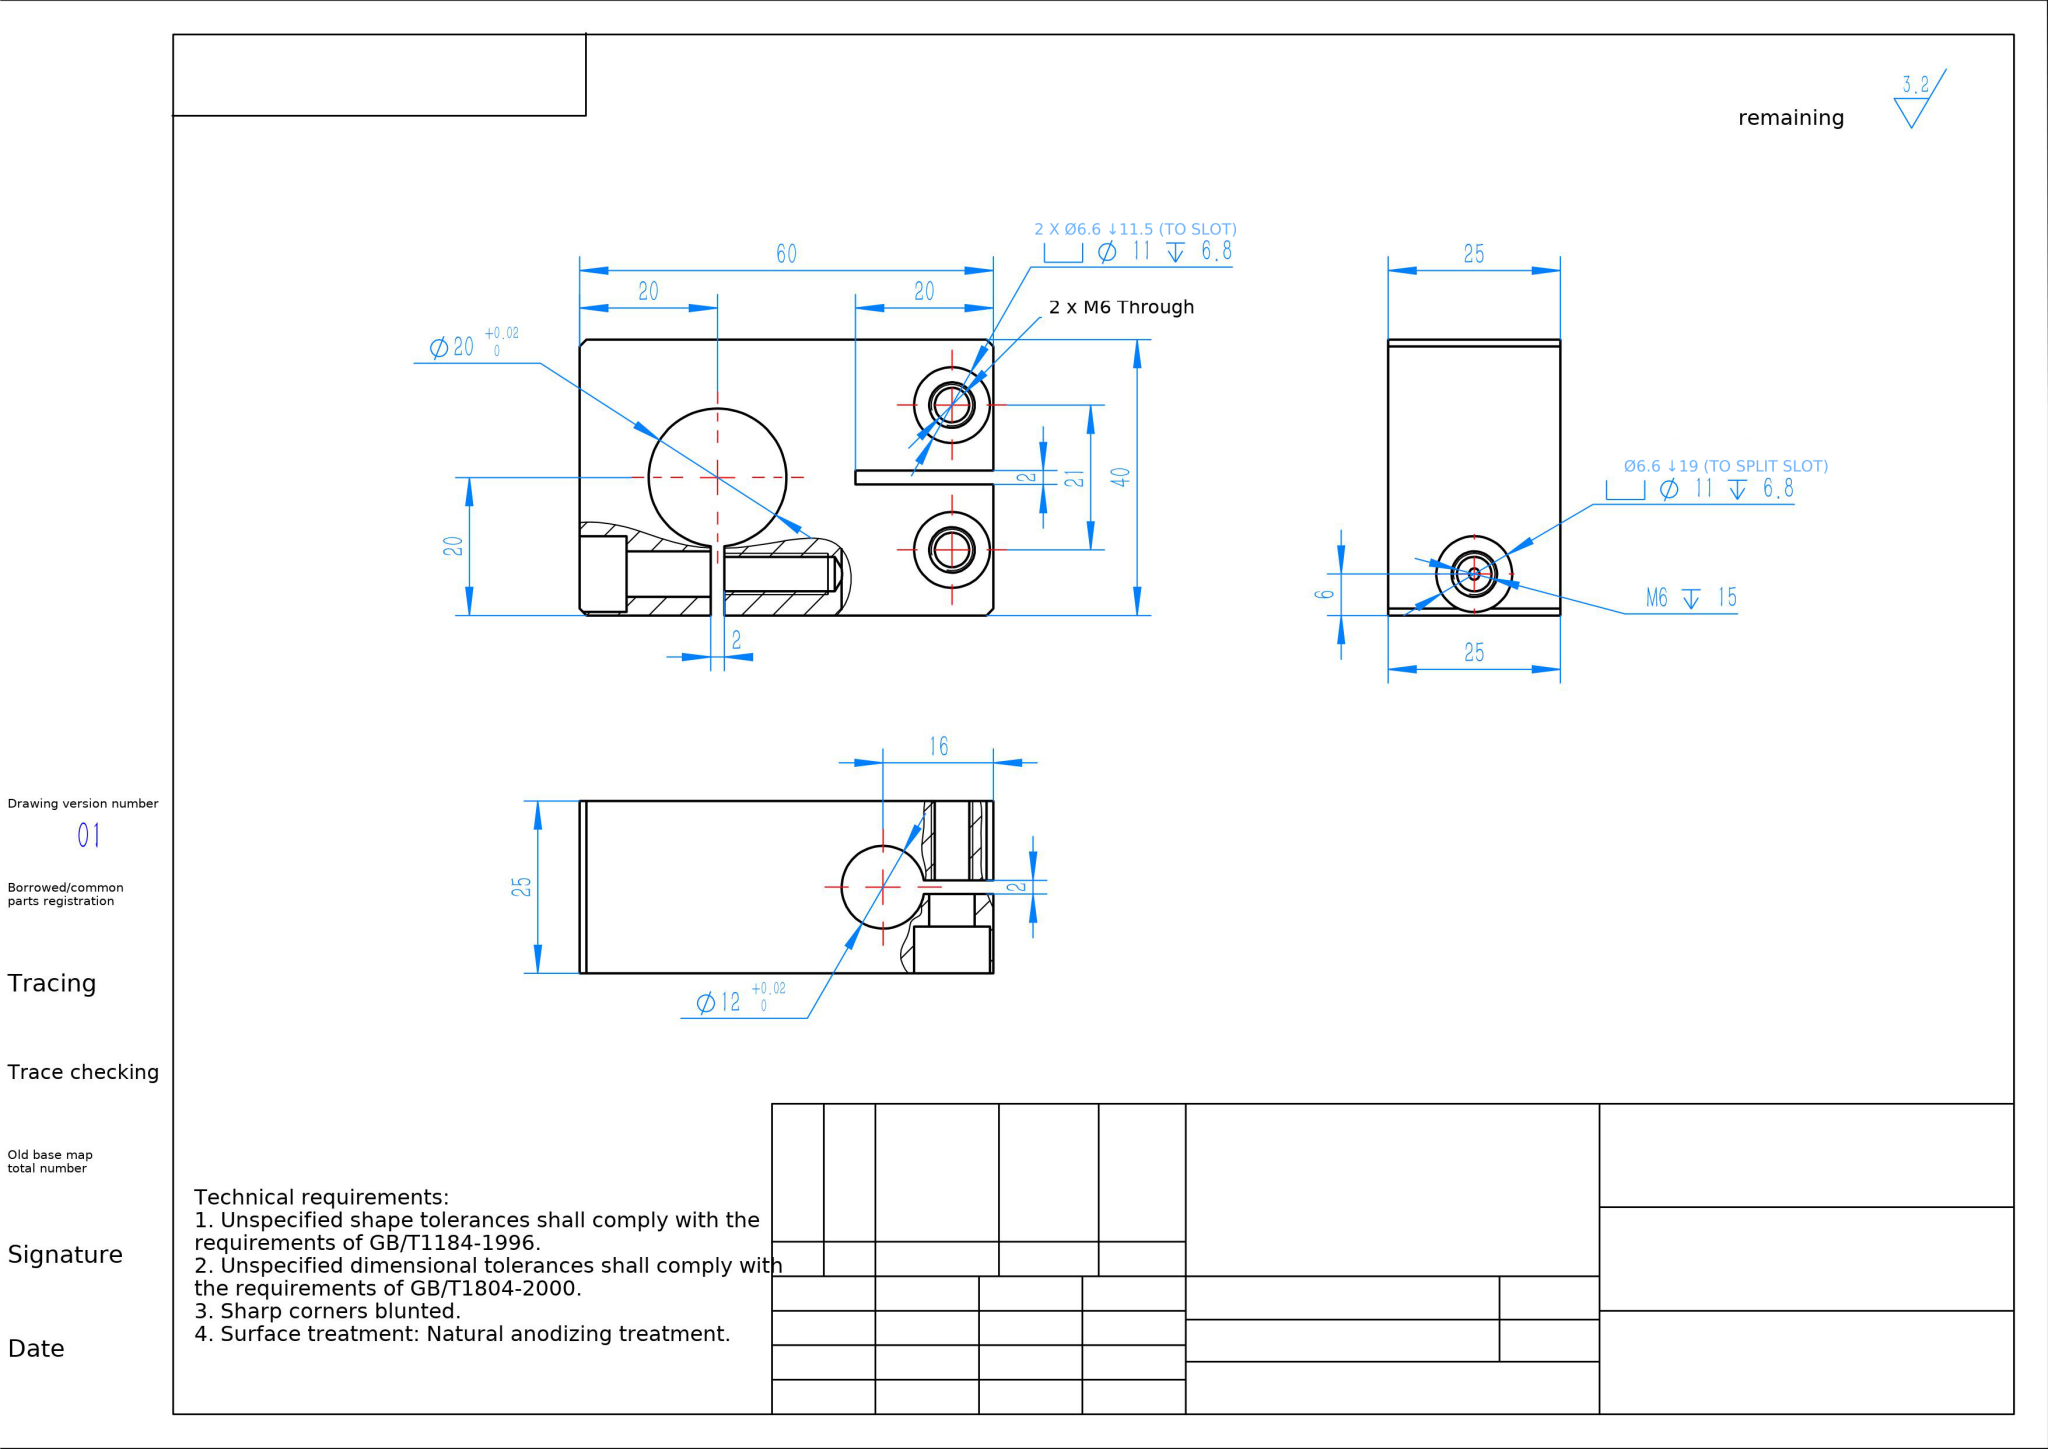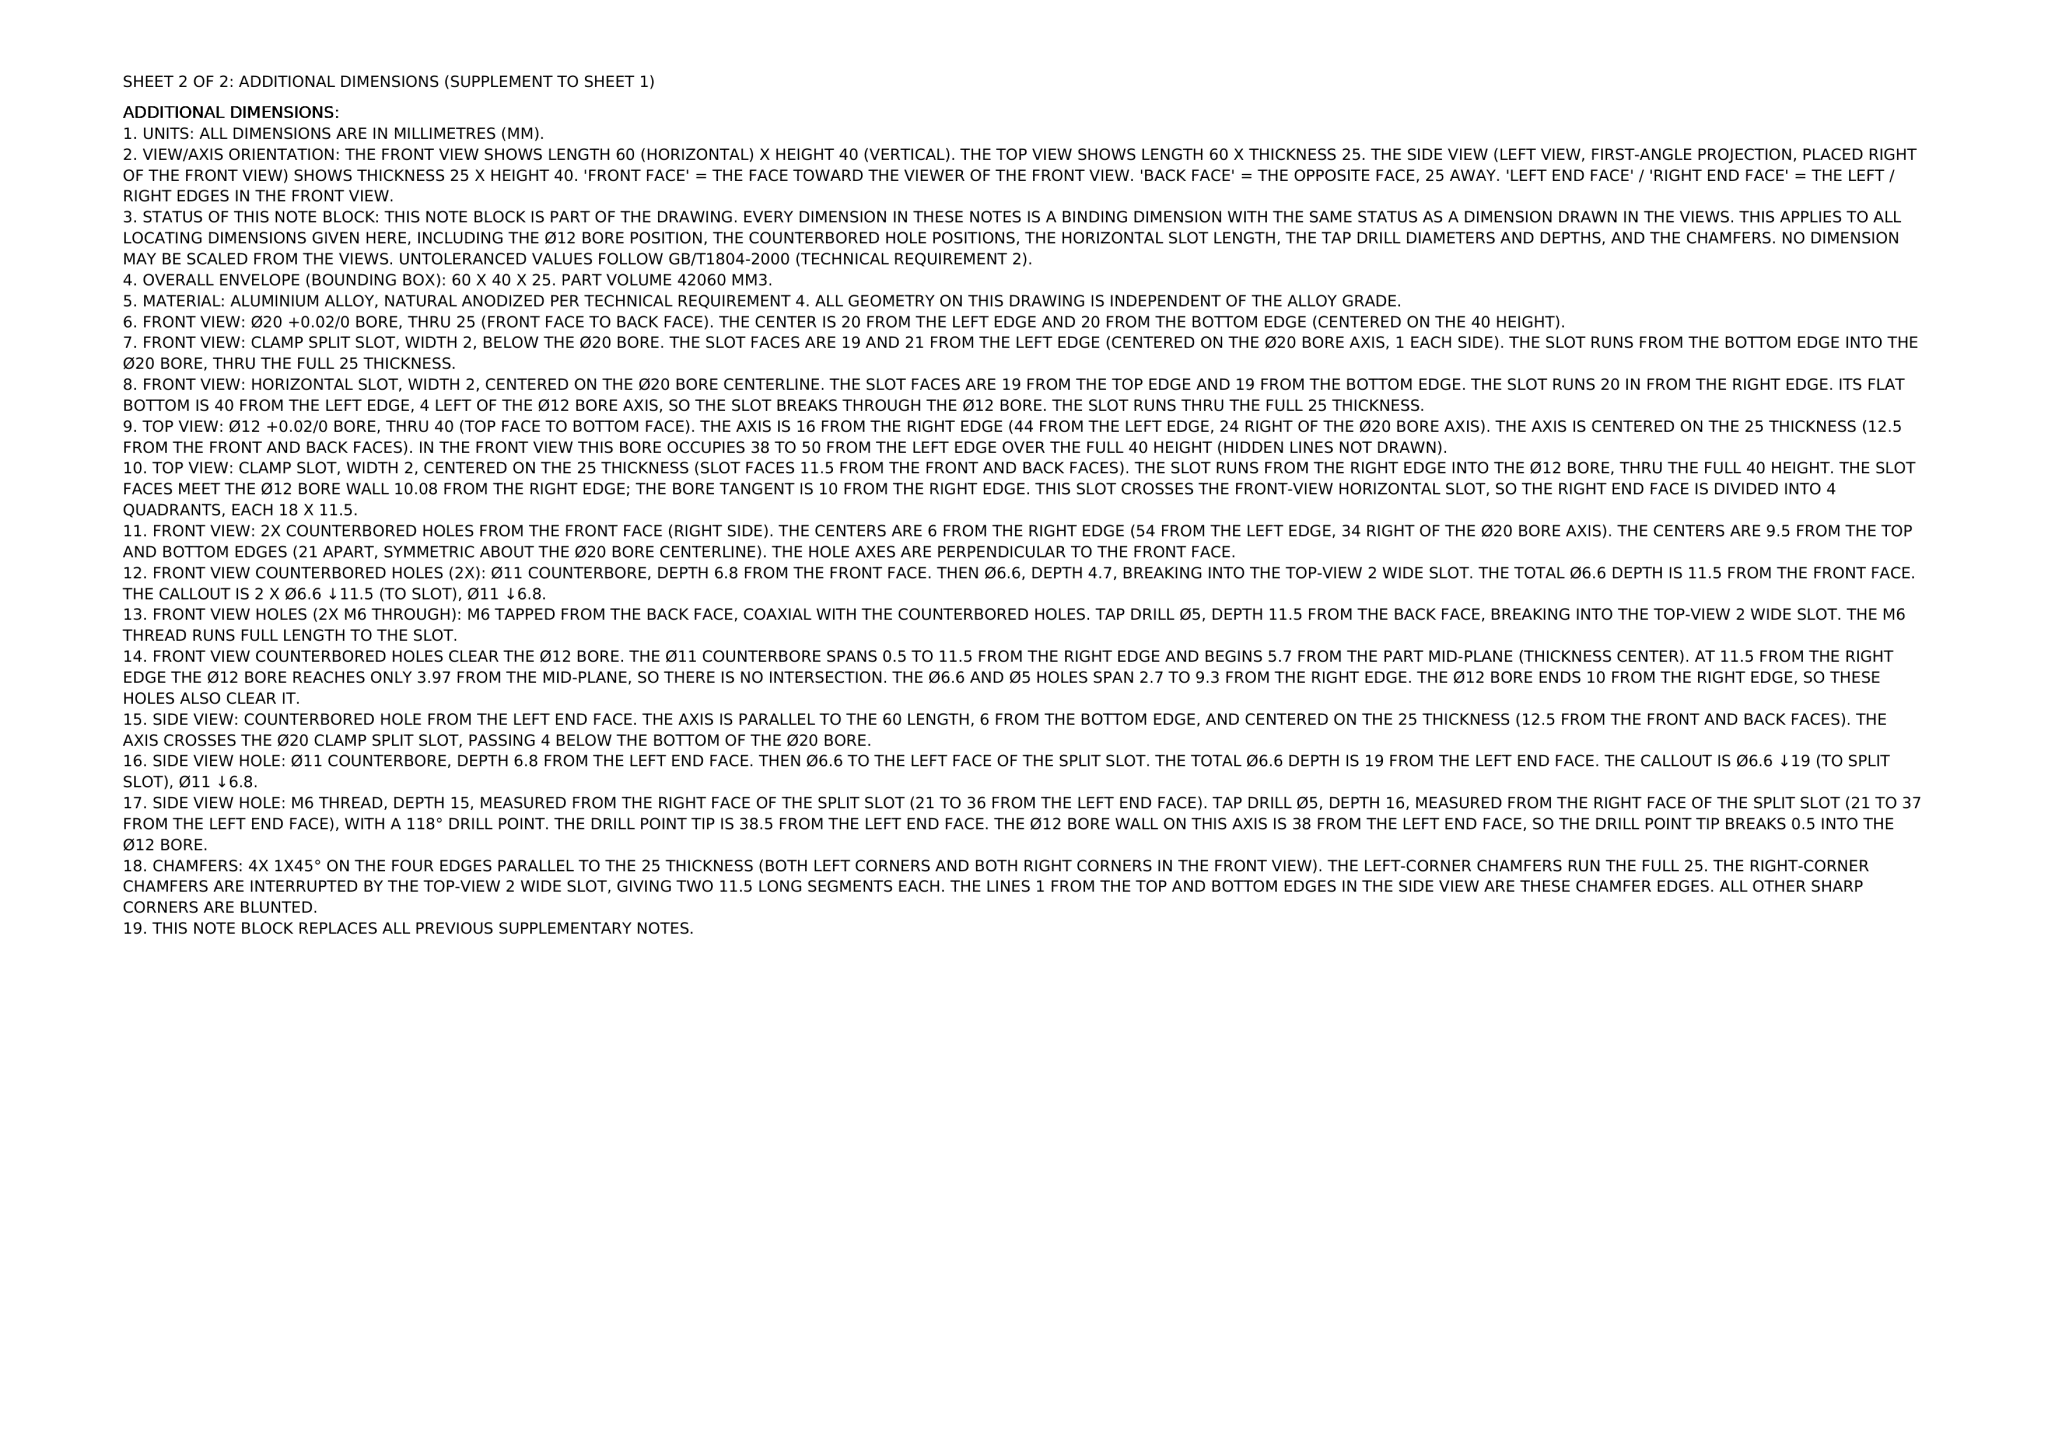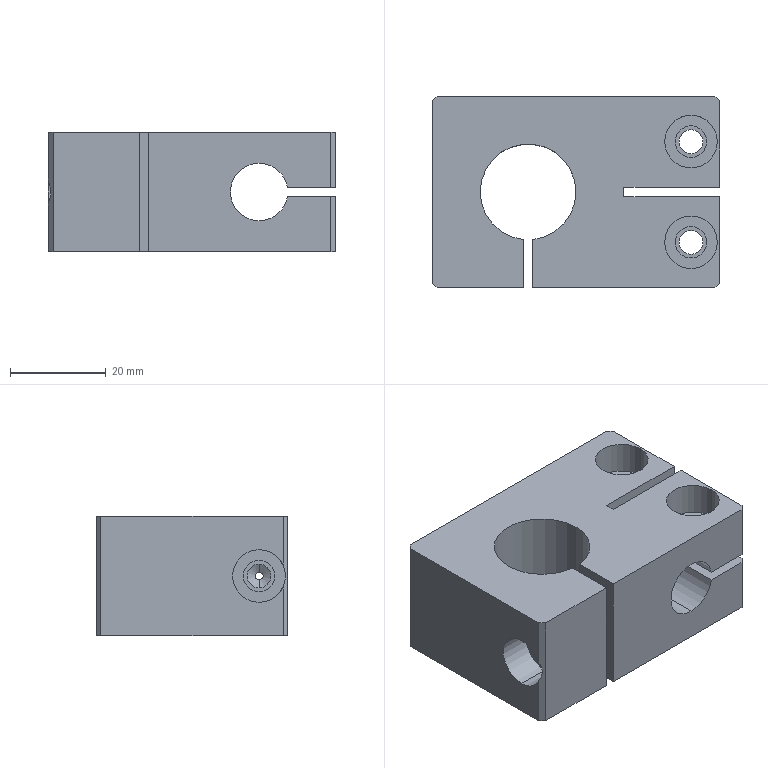Part | NX | mm | 1 solid | 59 faces | box 60 x 40 x 25 mm | volume 42060 mm3 | plane 31 | cylinder 26 | cone 2 | commonest cylinder face diameters 5 x6 6.6 x6 11 x6 12 x5 20 x3